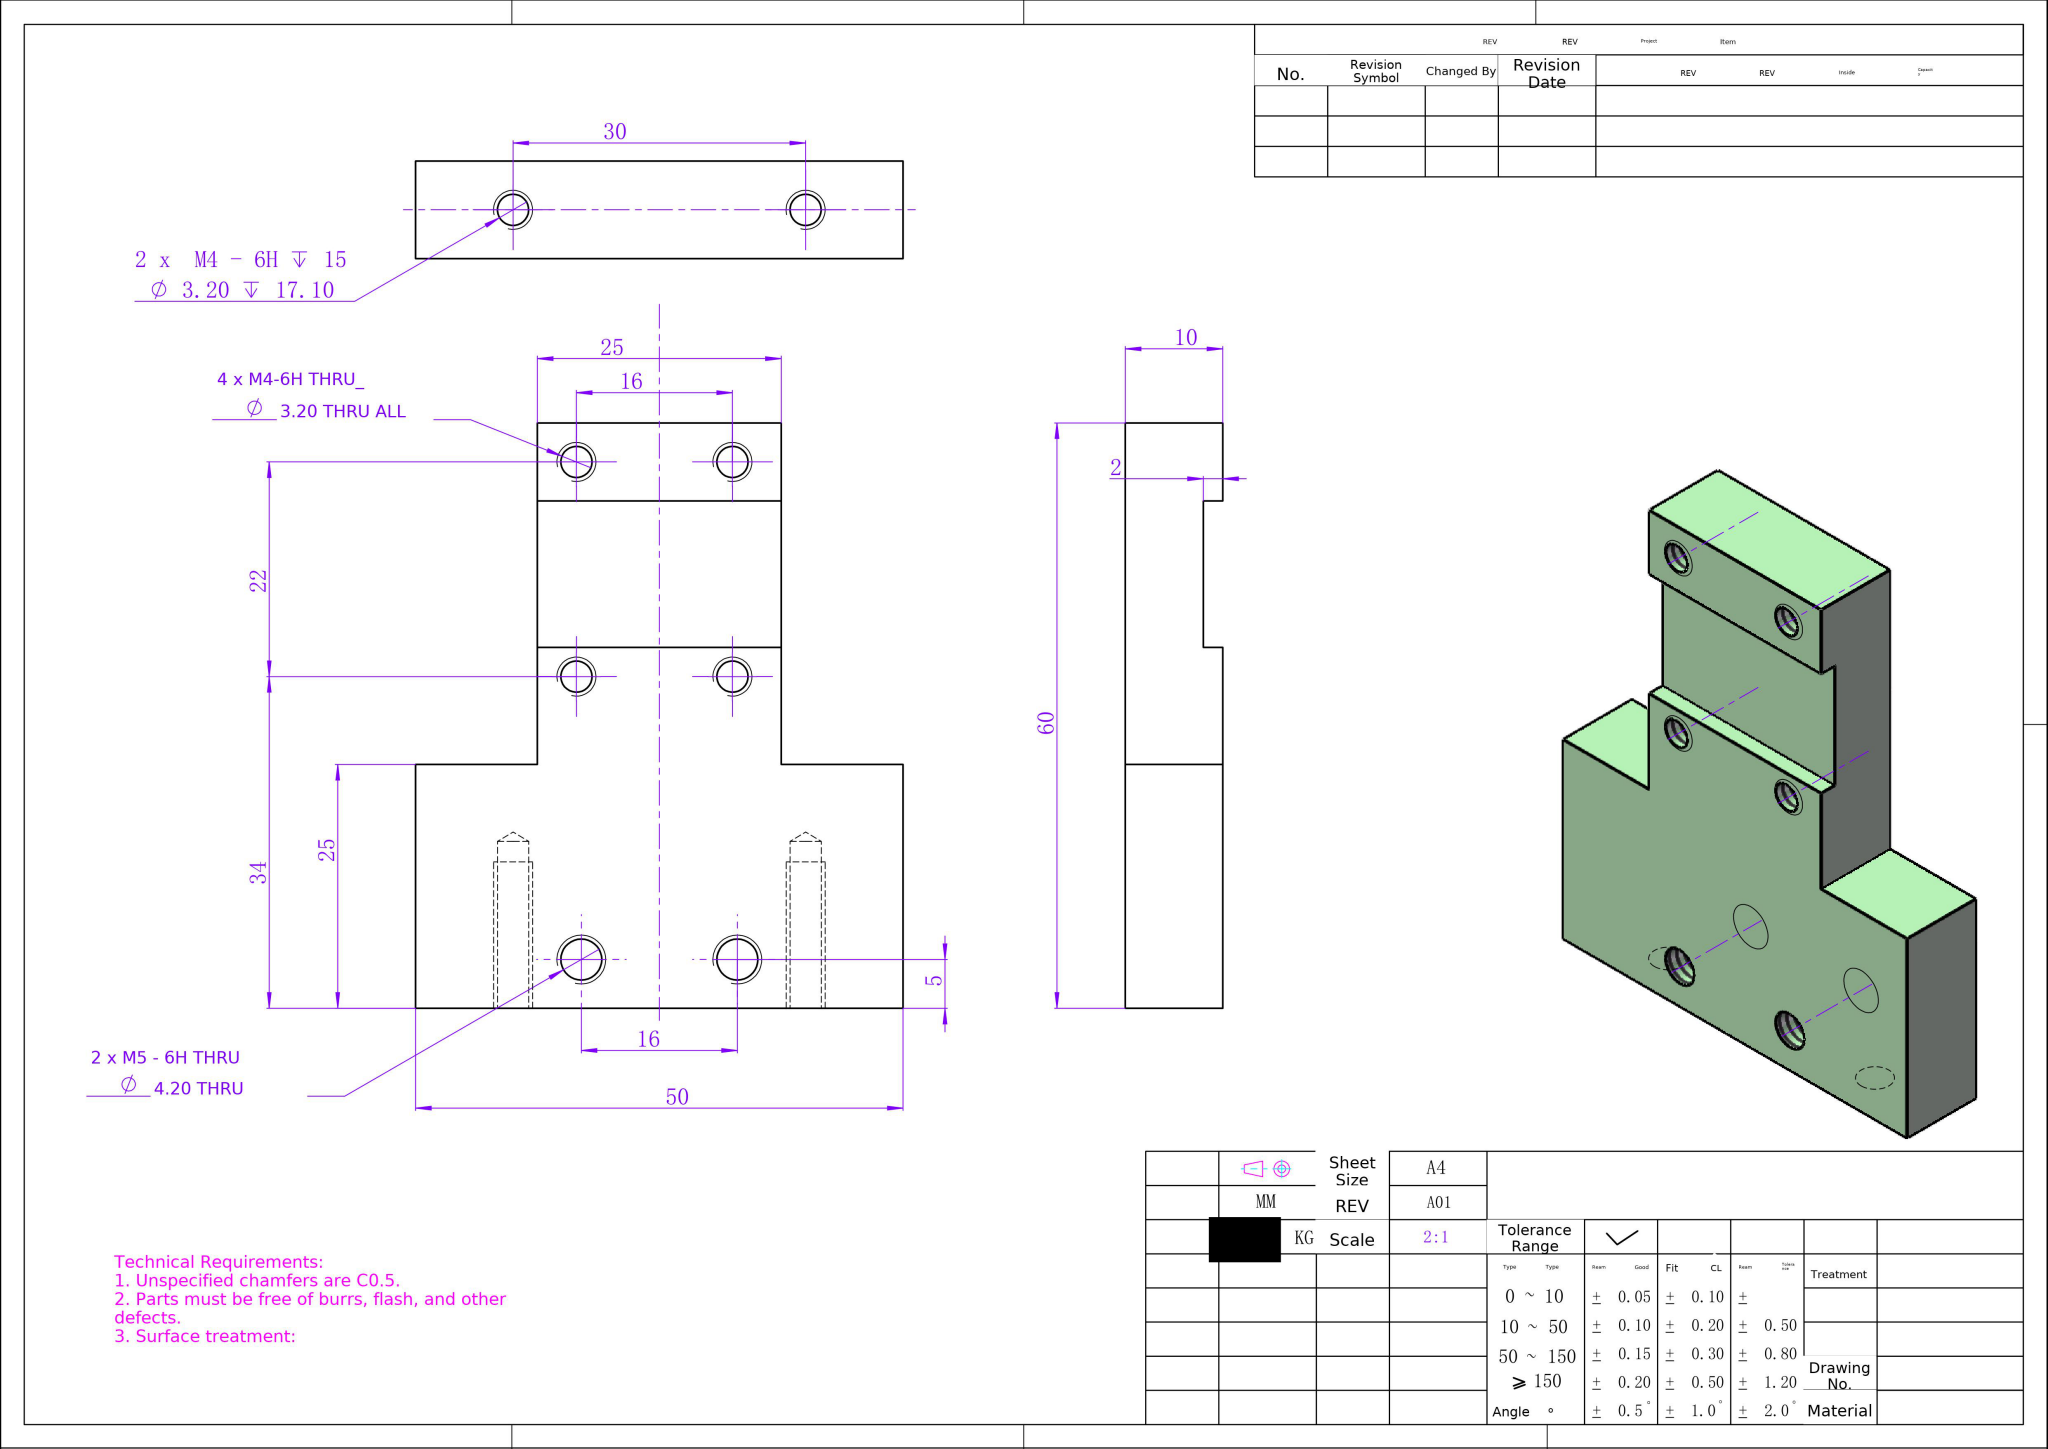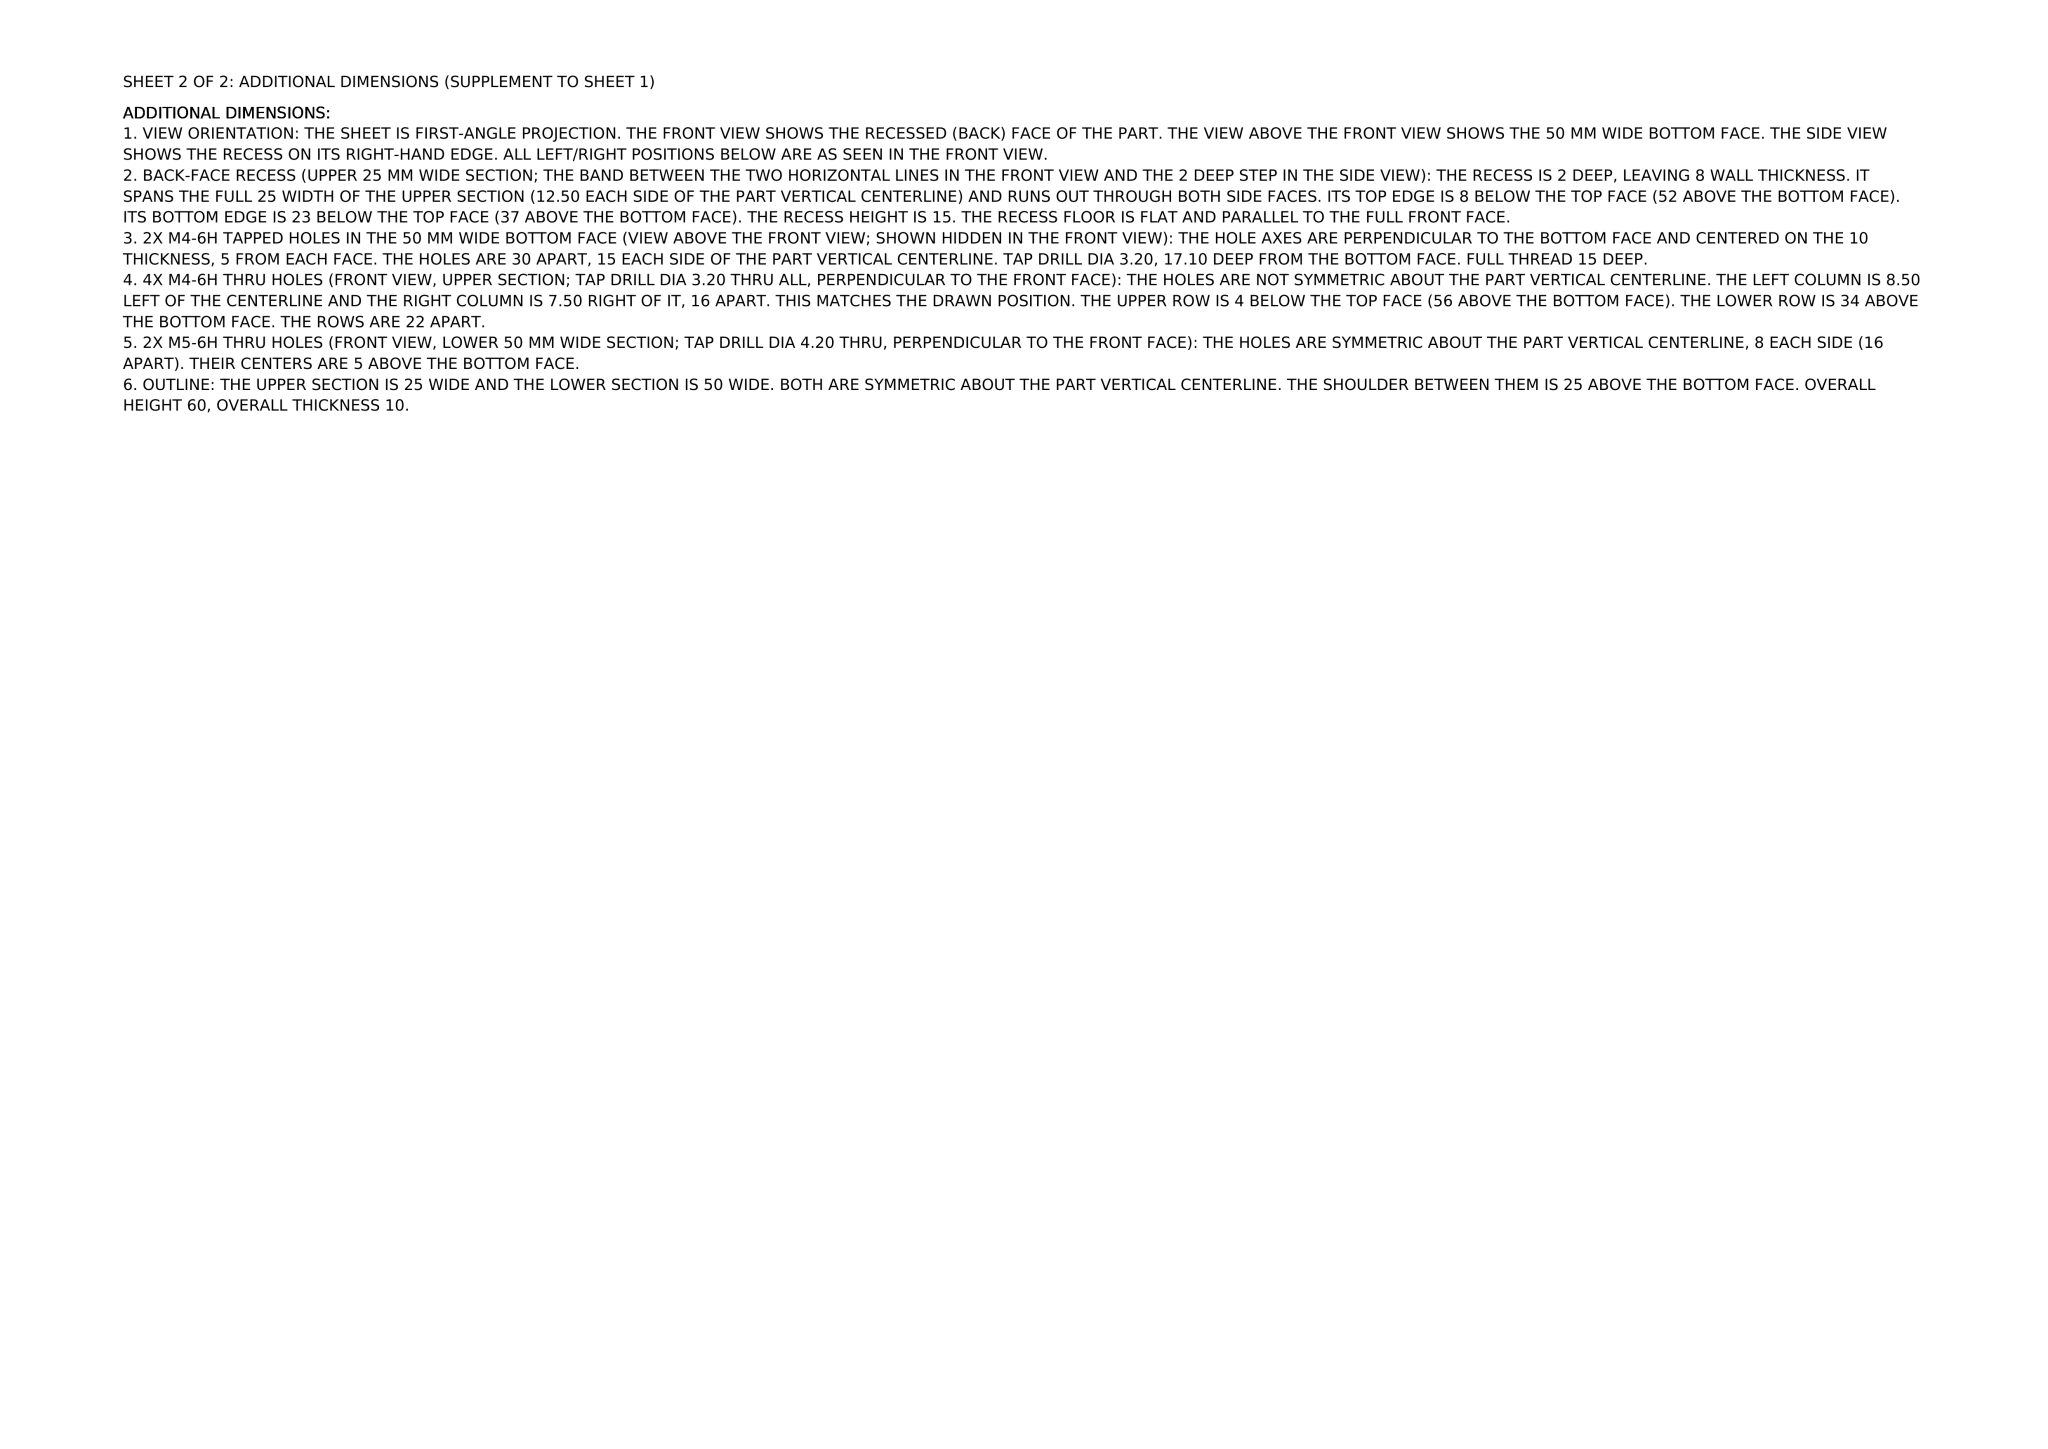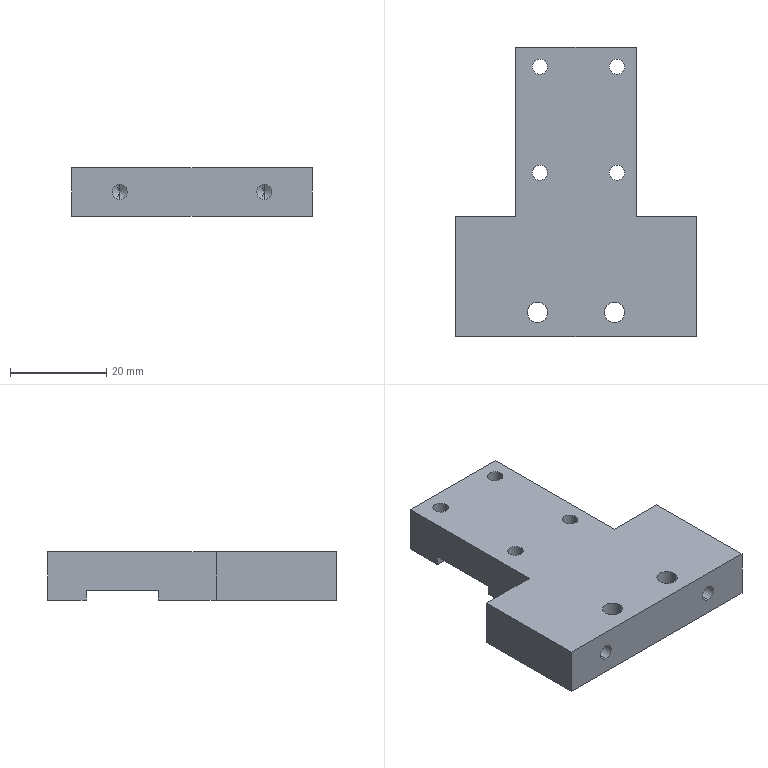Part | NX | mm | L-Shaped Six-Bore Mounting Bracket 60mm | 1 solid | 34 faces | box 50 x 60 x 10 mm | volume 19621 mm3 | cylinder 16 | plane 14 | cone 4 | commonest cylinder face diameters 3.2 x12 4.2 x4